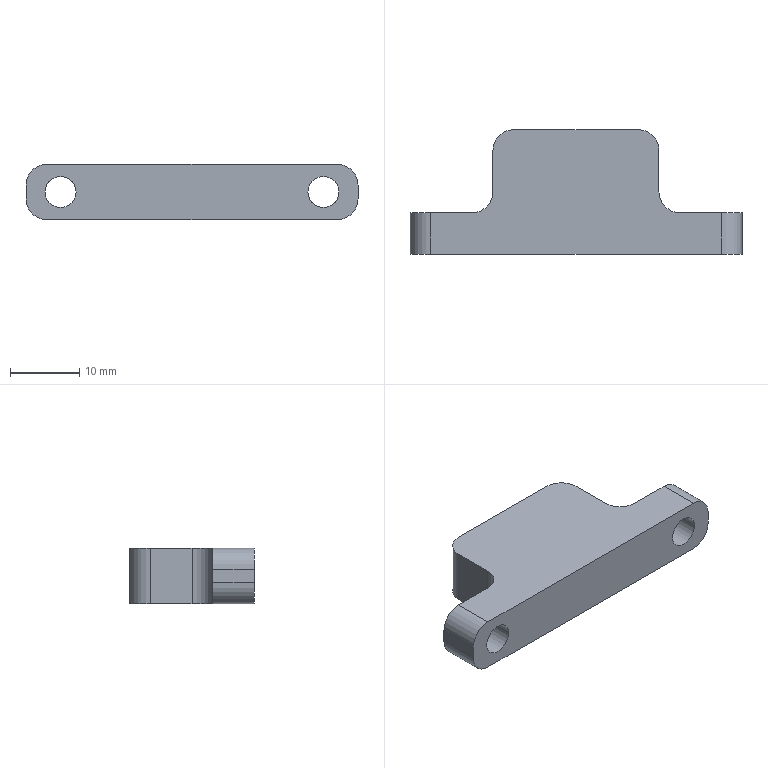CAM job | Mastercam | mm | 10 operations | part box 48 x 18 x 8
1. Facing | 24 - 100 平铣刀
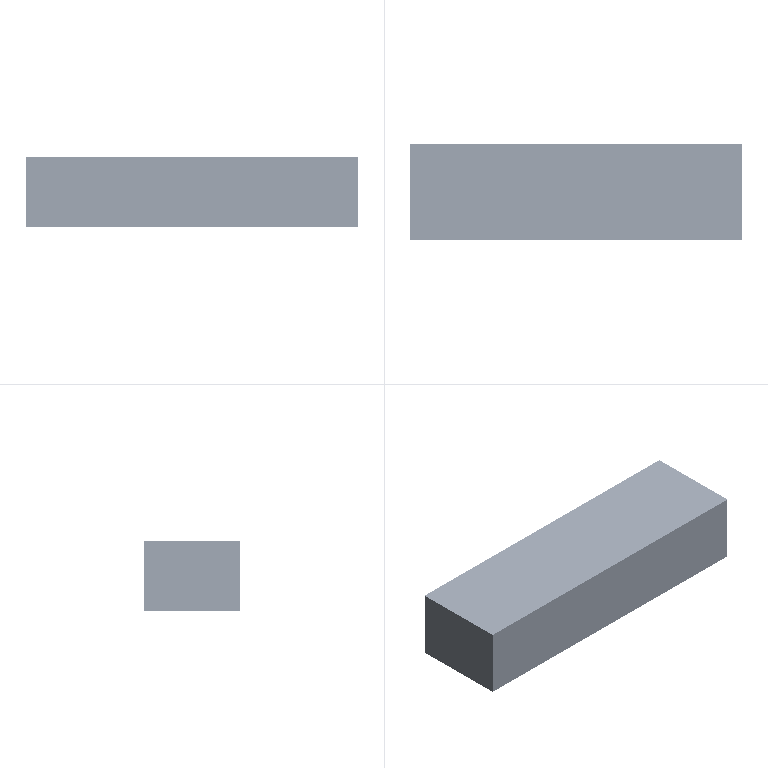2. 3D High Speed (Dynamic OptiRough) | 10 - 10 平铣刀
3. Surface Finish Flowline | 9 - 8 圆鼻铣刀
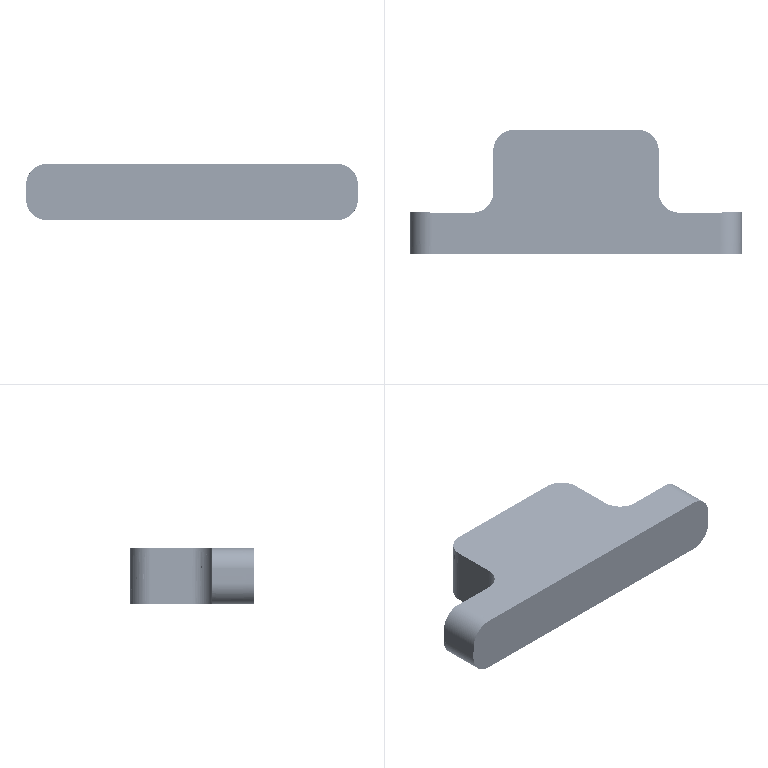4. Contour (2D) | 10 - 10 平铣刀
5. Contour (2D) | 10 - 10 平铣刀
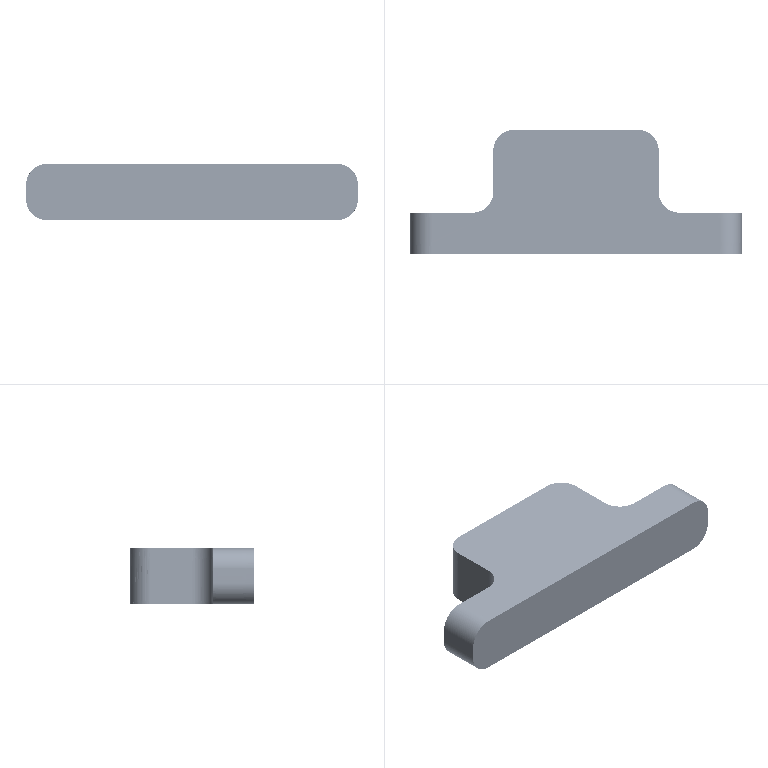6. Contour (2D) | 10 - 10 平铣刀
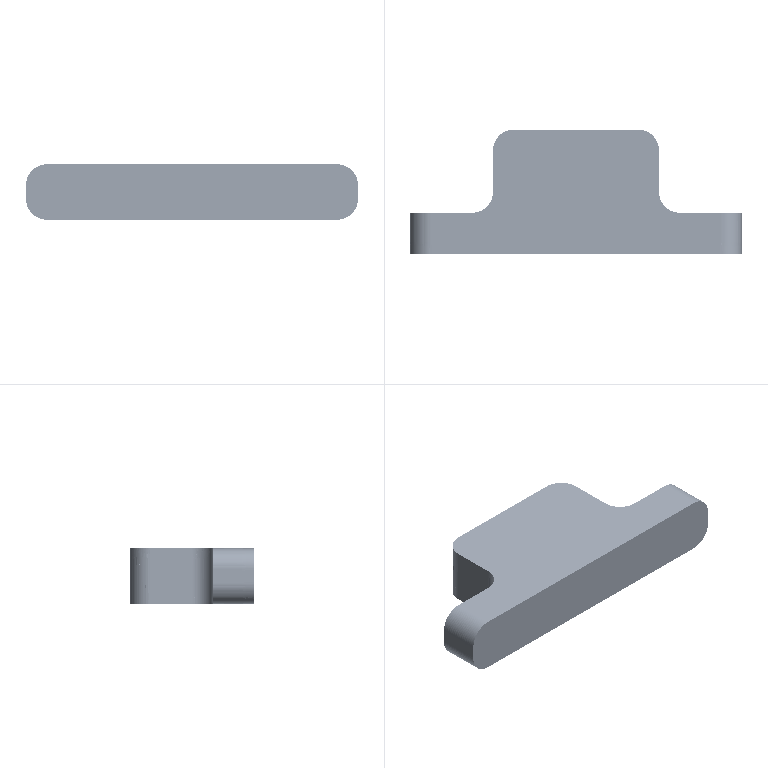7. Drill/Counterbore | 7 - 4 倒角刀
8. Deburr 5-axis | 5 - 4 球刀/圆鼻铣刀
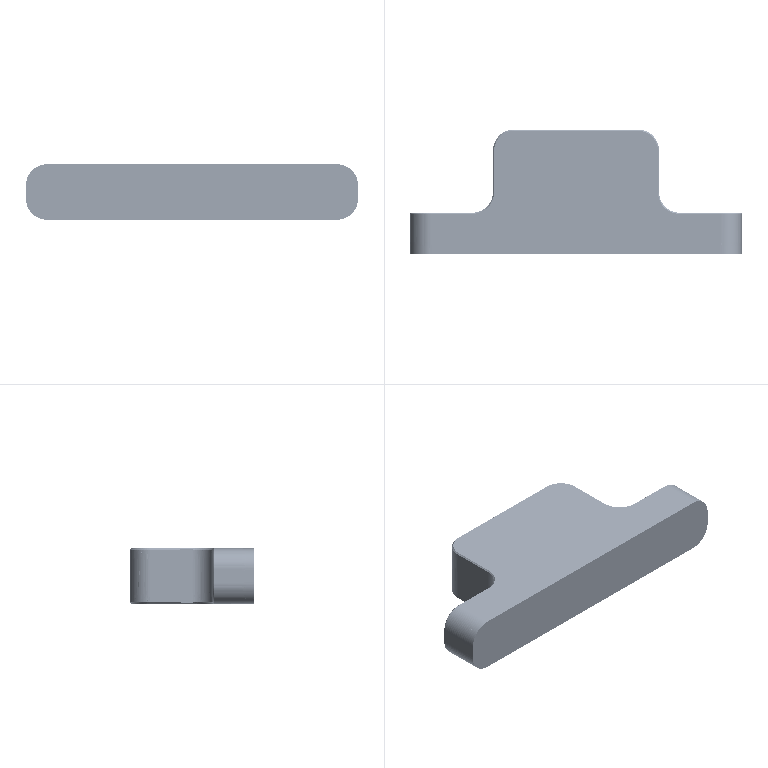9. Facing | 24 - 100 平铣刀
10. Contour (2D chamfer) | 7 - 4 倒角刀